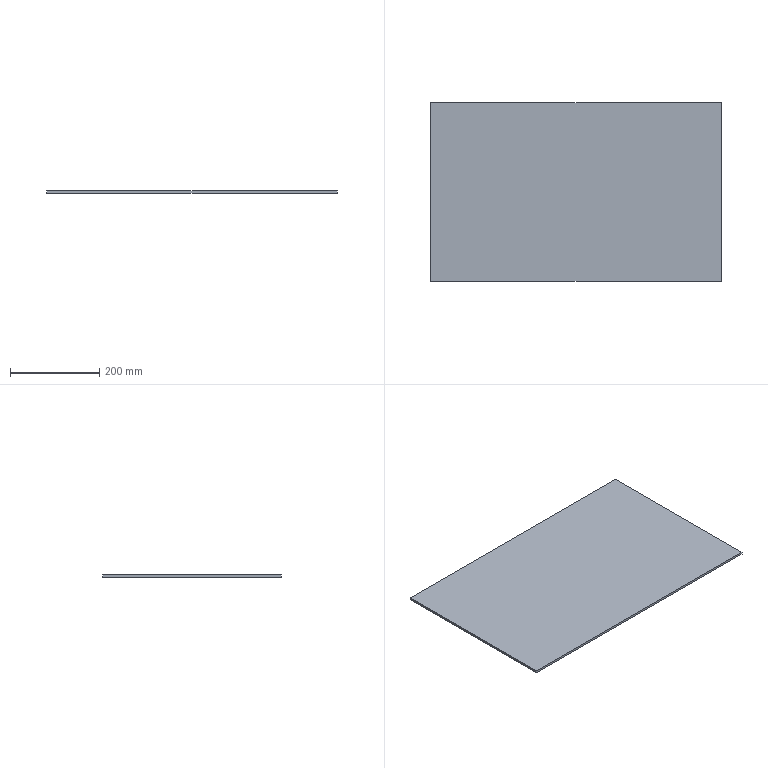Component | SolidWorks | AUTO-SpinDryWashing-01-03000003-1 | 1 solid | 6 faces | box 650 x 400 x 5 mm | volume 1300000 mm3 | plane 6 | material Glass
build123d program:
from build123d import *

# Parameters (mm, degrees)
SKETCH1_W           = 650
SKETCH1_H           = 400
BOSS_EXTRUDE1_DEPTH = 5


with BuildPart() as part:
    # Sketch1 → Boss-Extrude1 (new body)
    with BuildSketch(Plane.XY):
        Rectangle(SKETCH1_W, SKETCH1_H)
    extrude(amount=BOSS_EXTRUDE1_DEPTH)


solid = part.part

# Placed as in the assembly
solid = solid.moved(Location((0, 588, 55), (0, 0, 0)))
STEP:
#1=CARTESIAN_POINT('',(12.795,15.276,2.165));
#2=VERTEX_POINT('',#1);
#3=CARTESIAN_POINT('',(12.795,31.024,2.165));
#4=VERTEX_POINT('',#3);
#5=CARTESIAN_POINT('',(12.795,31.024,2.165));
#6=DIRECTION('',(0.,1.,0.));
#7=VECTOR('',#6,39.37);
#8=LINE('',#5,#7);
#9=EDGE_CURVE('',#2,#4,#8,.T.);
#10=ORIENTED_EDGE('',*,*,#9,.T.);
#11=CARTESIAN_POINT('',(12.795,31.024,2.362));
#12=VERTEX_POINT('',#11);
#13=CARTESIAN_POINT('',(12.795,31.024,2.362));
#14=DIRECTION('',(0.,0.,-1.));
#15=VECTOR('',#14,39.37);
#16=LINE('',#13,#15);
#17=EDGE_CURVE('',#12,#4,#16,.T.);
#18=ORIENTED_EDGE('',*,*,#17,.F.);
#19=CARTESIAN_POINT('',(12.795,15.276,2.362));
#20=VERTEX_POINT('',#19);
#21=CARTESIAN_POINT('',(12.795,31.024,2.362));
#22=DIRECTION('',(0.,1.,0.));
#23=VECTOR('',#22,39.37);
#24=LINE('',#21,#23);
#25=EDGE_CURVE('',#20,#12,#24,.T.);
#26=ORIENTED_EDGE('',*,*,#25,.F.);
#27=CARTESIAN_POINT('',(12.795,15.276,2.362));
#28=DIRECTION('',(0.,0.,-1.));
#29=VECTOR('',#28,39.37);
#30=LINE('',#27,#29);
#31=EDGE_CURVE('',#20,#2,#30,.T.);
#32=ORIENTED_EDGE('',*,*,#31,.T.);
#33=EDGE_LOOP('',(#10,#18,#26,#32));
#34=FACE_OUTER_BOUND('',#33,.T.);
#35=CARTESIAN_POINT('',(12.795,31.024,2.362));
#36=DIRECTION('',(-1.,0.,0.));
#37=DIRECTION('',(0.,0.,1.));
#38=AXIS2_PLACEMENT_3D('',#35,#36,#37);
#39=PLANE('',#38);
#40=ADVANCED_FACE('',(#34),#39,.F.);
#41=CARTESIAN_POINT('',(-12.795,31.024,2.165));
#42=VERTEX_POINT('',#41);
#43=CARTESIAN_POINT('',(-12.795,31.024,2.165));
#44=DIRECTION('',(-1.,0.,0.));
#45=VECTOR('',#44,39.37);
#46=LINE('',#43,#45);
#47=EDGE_CURVE('',#4,#42,#46,.T.);
#48=ORIENTED_EDGE('',*,*,#47,.T.);
#49=CARTESIAN_POINT('',(-12.795,31.024,2.362));
#50=VERTEX_POINT('',#49);
#51=CARTESIAN_POINT('',(-12.795,31.024,2.362));
#52=DIRECTION('',(0.,0.,-1.));
#53=VECTOR('',#52,39.37);
#54=LINE('',#51,#53);
#55=EDGE_CURVE('',#50,#42,#54,.T.);
#56=ORIENTED_EDGE('',*,*,#55,.F.);
#57=CARTESIAN_POINT('',(-12.795,31.024,2.362));
#58=DIRECTION('',(-1.,0.,0.));
#59=VECTOR('',#58,39.37);
#60=LINE('',#57,#59);
#61=EDGE_CURVE('',#12,#50,#60,.T.);
#62=ORIENTED_EDGE('',*,*,#61,.F.);
#63=ORIENTED_EDGE('',*,*,#17,.T.);
#64=EDGE_LOOP('',(#48,#56,#62,#63));
#65=FACE_OUTER_BOUND('',#64,.T.);
#66=CARTESIAN_POINT('',(-12.795,31.024,2.362));
#67=DIRECTION('',(0.,-1.,0.));
#68=DIRECTION('',(0.,0.,-1.));
#69=AXIS2_PLACEMENT_3D('',#66,#67,#68);
#70=PLANE('',#69);
#71=ADVANCED_FACE('',(#65),#70,.F.);
#72=CARTESIAN_POINT('',(-12.795,15.276,2.165));
#73=VERTEX_POINT('',#72);
#74=CARTESIAN_POINT('',(-12.795,31.024,2.165));
#75=DIRECTION('',(0.,-1.,0.));
#76=VECTOR('',#75,39.37);
#77=LINE('',#74,#76);
#78=EDGE_CURVE('',#42,#73,#77,.T.);
#79=ORIENTED_EDGE('',*,*,#78,.T.);
#80=CARTESIAN_POINT('',(-12.795,15.276,2.362));
#81=VERTEX_POINT('',#80);
#82=CARTESIAN_POINT('',(-12.795,15.276,2.362));
#83=DIRECTION('',(0.,0.,-1.));
#84=VECTOR('',#83,39.37);
#85=LINE('',#82,#84);
#86=EDGE_CURVE('',#81,#73,#85,.T.);
#87=ORIENTED_EDGE('',*,*,#86,.F.);
#88=CARTESIAN_POINT('',(-12.795,31.024,2.362));
#89=DIRECTION('',(0.,-1.,0.));
#90=VECTOR('',#89,39.37);
#91=LINE('',#88,#90);
#92=EDGE_CURVE('',#50,#81,#91,.T.);
#93=ORIENTED_EDGE('',*,*,#92,.F.);
#94=ORIENTED_EDGE('',*,*,#55,.T.);
#95=EDGE_LOOP('',(#79,#87,#93,#94));
#96=FACE_OUTER_BOUND('',#95,.T.);
#97=CARTESIAN_POINT('',(-12.795,31.024,2.362));
#98=DIRECTION('',(1.,0.,0.));
#99=DIRECTION('',(-0.,1.,0.));
#100=AXIS2_PLACEMENT_3D('',#97,#98,#99);
#101=PLANE('',#100);
#102=ADVANCED_FACE('',(#96),#101,.F.);
#103=CARTESIAN_POINT('',(-12.795,15.276,2.165));
#104=DIRECTION('',(1.,0.,0.));
#105=VECTOR('',#104,39.37);
#106=LINE('',#103,#105);
#107=EDGE_CURVE('',#73,#2,#106,.T.);
#108=ORIENTED_EDGE('',*,*,#107,.T.);
#109=ORIENTED_EDGE('',*,*,#31,.F.);
#110=CARTESIAN_POINT('',(-12.795,15.276,2.362));
#111=DIRECTION('',(1.,0.,0.));
#112=VECTOR('',#111,39.37);
#113=LINE('',#110,#112);
#114=EDGE_CURVE('',#81,#20,#113,.T.);
#115=ORIENTED_EDGE('',*,*,#114,.F.);
#116=ORIENTED_EDGE('',*,*,#86,.T.);
#117=EDGE_LOOP('',(#108,#109,#115,#116));
#118=FACE_OUTER_BOUND('',#117,.T.);
#119=CARTESIAN_POINT('',(-12.795,15.276,2.362));
#120=DIRECTION('',(0.,1.,0.));
#121=DIRECTION('',(0.,0.,1.));
#122=AXIS2_PLACEMENT_3D('',#119,#120,#121);
#123=PLANE('',#122);
#124=ADVANCED_FACE('',(#118),#123,.F.);
#125=ORIENTED_EDGE('',*,*,#25,.T.);
#126=ORIENTED_EDGE('',*,*,#61,.T.);
#127=ORIENTED_EDGE('',*,*,#92,.T.);
#128=ORIENTED_EDGE('',*,*,#114,.T.);
#129=EDGE_LOOP('',(#125,#126,#127,#128));
#130=FACE_OUTER_BOUND('',#129,.T.);
#131=CARTESIAN_POINT('',(0.,23.15,2.362));
#132=DIRECTION('',(0.,0.,1.));
#133=DIRECTION('',(1.,0.,0.));
#134=AXIS2_PLACEMENT_3D('',#131,#132,#133);
#135=PLANE('',#134);
#136=ADVANCED_FACE('',(#130),#135,.T.);
#137=ORIENTED_EDGE('',*,*,#9,.F.);
#138=ORIENTED_EDGE('',*,*,#107,.F.);
#139=ORIENTED_EDGE('',*,*,#78,.F.);
#140=ORIENTED_EDGE('',*,*,#47,.F.);
#141=EDGE_LOOP('',(#137,#138,#139,#140));
#142=FACE_OUTER_BOUND('',#141,.T.);
#143=CARTESIAN_POINT('',(0.,23.15,2.165));
#144=DIRECTION('',(0.,0.,1.));
#145=DIRECTION('',(1.,0.,0.));
#146=AXIS2_PLACEMENT_3D('',#143,#144,#145);
#147=PLANE('',#146);
#148=ADVANCED_FACE('',(#142),#147,.F.);
#149=CLOSED_SHELL('',(#40,#71,#102,#124,#136,#148));
#150=MANIFOLD_SOLID_BREP('',#149);
#151=CARTESIAN_POINT('',(0.,0.,0.));
#152=DIRECTION('',(0.,0.,1.));
#153=DIRECTION('',(1.,0.,0.));
#154=AXIS2_PLACEMENT_3D('',#151,#152,#153);
#155=(LENGTH_UNIT()NAMED_UNIT(*)SI_UNIT($,.METRE.));
#156=LENGTH_MEASURE_WITH_UNIT(LENGTH_MEASURE(0.0254),#155);
#157=DIMENSIONAL_EXPONENTS(1.,0.,0.,0.,0.,0.,0.);
#158=(CONVERSION_BASED_UNIT('',#156)LENGTH_UNIT()NAMED_UNIT(#157));
#159=UNCERTAINTY_MEASURE_WITH_UNIT(LENGTH_MEASURE(0.00001),#158,'','');
#160=(NAMED_UNIT(*)PLANE_ANGLE_UNIT()SI_UNIT($,.RADIAN.));
#161=(NAMED_UNIT(*)SI_UNIT($,.STERADIAN.)SOLID_ANGLE_UNIT());
#162=(GEOMETRIC_REPRESENTATION_CONTEXT(3)GLOBAL_UNCERTAINTY_ASSIGNED_CONTEXT((#159))GLOBAL_UNIT_ASSIGNED_CONTEXT((#158,#160,#161))REPRESENTATION_CONTEXT('',''));
#163=ADVANCED_BREP_SHAPE_REPRESENTATION('',(#150,#154),#162);
#164=COLOUR_RGB('',0.7922,0.8196,0.9333);
#165=FILL_AREA_STYLE_COLOUR('',#164);
#166=FILL_AREA_STYLE('',(#165));
#167=SURFACE_STYLE_FILL_AREA(#166);
#168=SURFACE_SIDE_STYLE('',(#167));
#169=SURFACE_STYLE_USAGE(.BOTH.,#168);
#170=PRESENTATION_STYLE_ASSIGNMENT((#169));
#171=STYLED_ITEM('',(#170),#150);
#172=(LENGTH_UNIT()NAMED_UNIT(*)SI_UNIT($,.METRE.));
#173=LENGTH_MEASURE_WITH_UNIT(LENGTH_MEASURE(0.0254),#172);
#174=DIMENSIONAL_EXPONENTS(1.,0.,0.,0.,0.,0.,0.);
#175=(CONVERSION_BASED_UNIT('',#173)LENGTH_UNIT()NAMED_UNIT(#174));
#176=UNCERTAINTY_MEASURE_WITH_UNIT(LENGTH_MEASURE(0.00001),#175,'','');
#177=(NAMED_UNIT(*)PLANE_ANGLE_UNIT()SI_UNIT($,.RADIAN.));
#178=(NAMED_UNIT(*)SI_UNIT($,.STERADIAN.)SOLID_ANGLE_UNIT());
#179=(GEOMETRIC_REPRESENTATION_CONTEXT(3)GLOBAL_UNCERTAINTY_ASSIGNED_CONTEXT((#176))GLOBAL_UNIT_ASSIGNED_CONTEXT((#175,#177,#178))REPRESENTATION_CONTEXT('',''));
#180=MECHANICAL_DESIGN_GEOMETRIC_PRESENTATION_REPRESENTATION('',(#171),#179);
#181=PRESENTATION_LAYER_ASSIGNMENT('','',(#171));